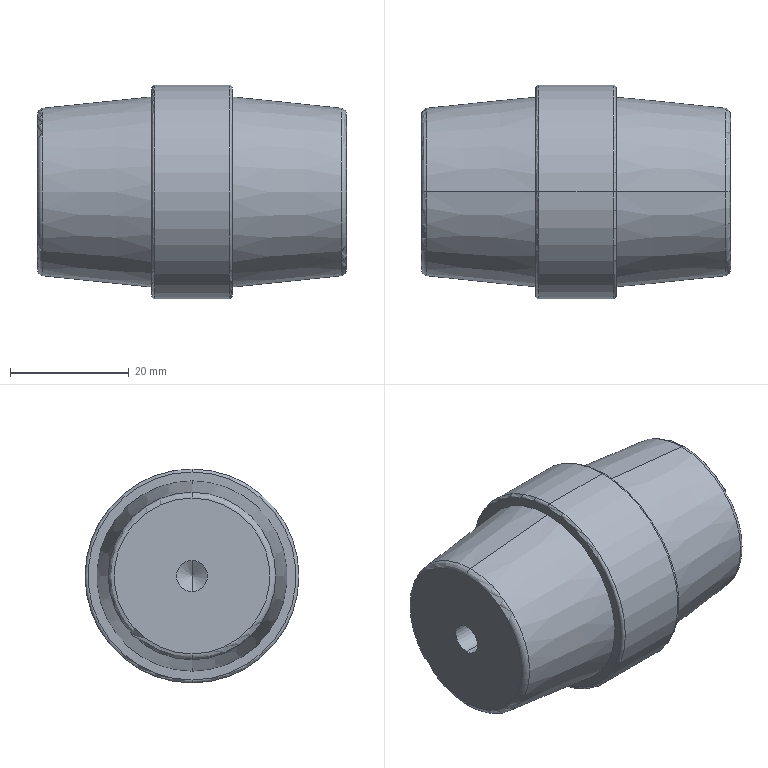Component | SolidWorks | InsulatorSYZ9-10Q100-1 | 1 solid | 26 faces | box 52 x 36 x 36 mm | volume 40423 mm3 | torus 8 | cone 8 | cylinder 6 | plane 4 | commonest cylinder face diameters 5.2 x4 36 x2
STEP:
#1=COLOUR_RGB('',0.7922,0.8196,0.9333);
#2=FILL_AREA_STYLE_COLOUR('',#1);
#3=FILL_AREA_STYLE('',(#2));
#4=SURFACE_STYLE_FILL_AREA(#3);
#5=SURFACE_SIDE_STYLE('',(#4));
#6=SURFACE_STYLE_USAGE(.BOTH.,#5);
#7=PRESENTATION_STYLE_ASSIGNMENT((#6));
#8=CARTESIAN_POINT('',(25.13,9.025,27.254));
#9=VERTEX_POINT('',#8);
#10=CARTESIAN_POINT('',(25.13,9.025,28.671));
#11=VERTEX_POINT('',#10);
#12=CARTESIAN_POINT('',(25.13,9.025,27.963));
#13=DIRECTION('',(1.,0.,0.));
#14=DIRECTION('',(0.,0.,1.));
#15=AXIS2_PLACEMENT_3D('',#12,#13,#14);
#16=CIRCLE('',#15,0.7087);
#17=EDGE_CURVE('',#9,#11,#16,.T.);
#18=ORIENTED_EDGE('',*,*,#17,.F.);
#19=CARTESIAN_POINT('',(25.11,9.025,27.274));
#20=VERTEX_POINT('',#19);
#21=CARTESIAN_POINT('',(25.13,9.025,27.274));
#22=DIRECTION('',(0.,1.,0.));
#23=DIRECTION('',(0.,0.,1.));
#24=AXIS2_PLACEMENT_3D('',#21,#22,#23);
#25=CIRCLE('',#24,0.01969);
#26=EDGE_CURVE('',#9,#20,#25,.T.);
#27=ORIENTED_EDGE('',*,*,#26,.T.);
#28=CARTESIAN_POINT('',(25.11,9.025,28.652));
#29=VERTEX_POINT('',#28);
#30=CARTESIAN_POINT('',(25.11,9.025,27.963));
#31=DIRECTION('',(-1.,0.,0.));
#32=DIRECTION('',(0.,0.,1.));
#33=AXIS2_PLACEMENT_3D('',#30,#31,#32);
#34=CIRCLE('',#33,0.689);
#35=EDGE_CURVE('',#29,#20,#34,.T.);
#36=ORIENTED_EDGE('',*,*,#35,.F.);
#37=CARTESIAN_POINT('',(25.13,9.025,28.652));
#38=DIRECTION('',(0.,-1.,0.));
#39=DIRECTION('',(0.,0.,-1.));
#40=AXIS2_PLACEMENT_3D('',#37,#38,#39);
#41=CIRCLE('',#40,0.01969);
#42=EDGE_CURVE('',#11,#29,#41,.T.);
#43=ORIENTED_EDGE('',*,*,#42,.F.);
#44=EDGE_LOOP('',(#18,#27,#36,#43));
#45=FACE_OUTER_BOUND('',#44,.T.);
#46=CARTESIAN_POINT('',(25.13,9.025,27.963));
#47=DIRECTION('',(-1.,0.,0.));
#48=DIRECTION('',(0.,0.,1.));
#49=AXIS2_PLACEMENT_3D('',#46,#47,#48);
#50=TOROIDAL_SURFACE('',#49,0.689,0.01969);
#51=ADVANCED_FACE('',(#45),#50,.T.);
#52=CARTESIAN_POINT('',(25.622,9.025,28.671));
#53=VERTEX_POINT('',#52);
#54=CARTESIAN_POINT('',(25.622,9.025,27.254));
#55=VERTEX_POINT('',#54);
#56=CARTESIAN_POINT('',(25.622,9.025,27.963));
#57=DIRECTION('',(-1.,0.,0.));
#58=DIRECTION('',(0.,0.,-1.));
#59=AXIS2_PLACEMENT_3D('',#56,#57,#58);
#60=CIRCLE('',#59,0.7087);
#61=EDGE_CURVE('',#53,#55,#60,.T.);
#62=ORIENTED_EDGE('',*,*,#61,.F.);
#63=CARTESIAN_POINT('',(25.642,9.025,28.652));
#64=VERTEX_POINT('',#63);
#65=CARTESIAN_POINT('',(25.622,9.025,28.652));
#66=DIRECTION('',(0.,1.,-0.));
#67=DIRECTION('',(0.,0.,1.));
#68=AXIS2_PLACEMENT_3D('',#65,#66,#67);
#69=CIRCLE('',#68,0.01969);
#70=EDGE_CURVE('',#53,#64,#69,.T.);
#71=ORIENTED_EDGE('',*,*,#70,.T.);
#72=CARTESIAN_POINT('',(25.642,9.025,27.274));
#73=VERTEX_POINT('',#72);
#74=CARTESIAN_POINT('',(25.642,9.025,27.963));
#75=DIRECTION('',(1.,0.,0.));
#76=DIRECTION('',(0.,0.,-1.));
#77=AXIS2_PLACEMENT_3D('',#74,#75,#76);
#78=CIRCLE('',#77,0.689);
#79=EDGE_CURVE('',#73,#64,#78,.T.);
#80=ORIENTED_EDGE('',*,*,#79,.F.);
#81=CARTESIAN_POINT('',(25.622,9.025,27.274));
#82=DIRECTION('',(0.,-1.,0.));
#83=DIRECTION('',(0.,0.,-1.));
#84=AXIS2_PLACEMENT_3D('',#81,#82,#83);
#85=CIRCLE('',#84,0.01969);
#86=EDGE_CURVE('',#55,#73,#85,.T.);
#87=ORIENTED_EDGE('',*,*,#86,.F.);
#88=EDGE_LOOP('',(#62,#71,#80,#87));
#89=FACE_OUTER_BOUND('',#88,.T.);
#90=CARTESIAN_POINT('',(25.622,9.025,27.963));
#91=DIRECTION('',(1.,0.,0.));
#92=DIRECTION('',(0.,0.,-1.));
#93=AXIS2_PLACEMENT_3D('',#90,#91,#92);
#94=TOROIDAL_SURFACE('',#93,0.689,0.01969);
#95=ADVANCED_FACE('',(#89),#94,.T.);
#96=CARTESIAN_POINT('',(24.388,9.025,27.408));
#97=VERTEX_POINT('',#96);
#98=CARTESIAN_POINT('',(24.388,9.025,28.517));
#99=VERTEX_POINT('',#98);
#100=CARTESIAN_POINT('',(24.388,9.025,27.963));
#101=DIRECTION('',(1.,0.,0.));
#102=DIRECTION('',(0.,0.,1.));
#103=AXIS2_PLACEMENT_3D('',#100,#101,#102);
#104=CIRCLE('',#103,0.5548);
#105=EDGE_CURVE('',#97,#99,#104,.T.);
#106=ORIENTED_EDGE('',*,*,#105,.F.);
#107=CARTESIAN_POINT('',(24.353,9.025,27.447));
#108=VERTEX_POINT('',#107);
#109=CARTESIAN_POINT('',(24.392,9.025,27.447));
#110=DIRECTION('',(0.,1.,0.));
#111=DIRECTION('',(0.,0.,1.));
#112=AXIS2_PLACEMENT_3D('',#109,#110,#111);
#113=CIRCLE('',#112,0.03937);
#114=EDGE_CURVE('',#97,#108,#113,.T.);
#115=ORIENTED_EDGE('',*,*,#114,.T.);
#116=CARTESIAN_POINT('',(24.353,9.025,28.478));
#117=VERTEX_POINT('',#116);
#118=CARTESIAN_POINT('',(24.353,9.025,27.963));
#119=DIRECTION('',(-1.,0.,0.));
#120=DIRECTION('',(0.,0.,1.));
#121=AXIS2_PLACEMENT_3D('',#118,#119,#120);
#122=CIRCLE('',#121,0.5157);
#123=EDGE_CURVE('',#117,#108,#122,.T.);
#124=ORIENTED_EDGE('',*,*,#123,.F.);
#125=CARTESIAN_POINT('',(24.392,9.025,28.478));
#126=DIRECTION('',(0.,-1.,0.));
#127=DIRECTION('',(0.,0.,-1.));
#128=AXIS2_PLACEMENT_3D('',#125,#126,#127);
#129=CIRCLE('',#128,0.03937);
#130=EDGE_CURVE('',#99,#117,#129,.T.);
#131=ORIENTED_EDGE('',*,*,#130,.F.);
#132=EDGE_LOOP('',(#106,#115,#124,#131));
#133=FACE_OUTER_BOUND('',#132,.T.);
#134=CARTESIAN_POINT('',(24.392,9.025,27.963));
#135=DIRECTION('',(-1.,0.,0.));
#136=DIRECTION('',(0.,0.,1.));
#137=AXIS2_PLACEMENT_3D('',#134,#135,#136);
#138=TOROIDAL_SURFACE('',#137,0.5157,0.03937);
#139=ADVANCED_FACE('',(#133),#138,.T.);
#140=CARTESIAN_POINT('',(26.364,9.025,28.517));
#141=VERTEX_POINT('',#140);
#142=CARTESIAN_POINT('',(26.364,9.025,27.408));
#143=VERTEX_POINT('',#142);
#144=CARTESIAN_POINT('',(26.364,9.025,27.963));
#145=DIRECTION('',(-1.,0.,0.));
#146=DIRECTION('',(0.,0.,-1.));
#147=AXIS2_PLACEMENT_3D('',#144,#145,#146);
#148=CIRCLE('',#147,0.5548);
#149=EDGE_CURVE('',#141,#143,#148,.T.);
#150=ORIENTED_EDGE('',*,*,#149,.F.);
#151=CARTESIAN_POINT('',(26.4,9.025,28.478));
#152=VERTEX_POINT('',#151);
#153=CARTESIAN_POINT('',(26.36,9.025,28.478));
#154=DIRECTION('',(0.,1.,-0.));
#155=DIRECTION('',(0.,0.,1.));
#156=AXIS2_PLACEMENT_3D('',#153,#154,#155);
#157=CIRCLE('',#156,0.03937);
#158=EDGE_CURVE('',#141,#152,#157,.T.);
#159=ORIENTED_EDGE('',*,*,#158,.T.);
#160=CARTESIAN_POINT('',(26.4,9.025,27.447));
#161=VERTEX_POINT('',#160);
#162=CARTESIAN_POINT('',(26.4,9.025,27.963));
#163=DIRECTION('',(1.,0.,0.));
#164=DIRECTION('',(0.,0.,-1.));
#165=AXIS2_PLACEMENT_3D('',#162,#163,#164);
#166=CIRCLE('',#165,0.5157);
#167=EDGE_CURVE('',#161,#152,#166,.T.);
#168=ORIENTED_EDGE('',*,*,#167,.F.);
#169=CARTESIAN_POINT('',(26.36,9.025,27.447));
#170=DIRECTION('',(0.,-1.,0.));
#171=DIRECTION('',(0.,0.,-1.));
#172=AXIS2_PLACEMENT_3D('',#169,#170,#171);
#173=CIRCLE('',#172,0.03937);
#174=EDGE_CURVE('',#143,#161,#173,.T.);
#175=ORIENTED_EDGE('',*,*,#174,.F.);
#176=EDGE_LOOP('',(#150,#159,#168,#175));
#177=FACE_OUTER_BOUND('',#176,.T.);
#178=CARTESIAN_POINT('',(26.36,9.025,27.963));
#179=DIRECTION('',(1.,0.,0.));
#180=DIRECTION('',(0.,0.,-1.));
#181=AXIS2_PLACEMENT_3D('',#178,#179,#180);
#182=TOROIDAL_SURFACE('',#181,0.5157,0.03937);
#183=ADVANCED_FACE('',(#177),#182,.T.);
#184=CARTESIAN_POINT('',(25.927,9.025,28.065));
#185=VERTEX_POINT('',#184);
#186=CARTESIAN_POINT('',(25.927,9.025,27.86));
#187=VERTEX_POINT('',#186);
#188=CARTESIAN_POINT('',(25.927,9.025,27.963));
#189=DIRECTION('',(1.,0.,0.));
#190=DIRECTION('',(0.,0.,-1.));
#191=AXIS2_PLACEMENT_3D('',#188,#189,#190);
#192=CIRCLE('',#191,0.1024);
#193=EDGE_CURVE('',#185,#187,#192,.T.);
#194=ORIENTED_EDGE('',*,*,#193,.F.);
#195=CARTESIAN_POINT('',(26.4,9.025,28.065));
#196=VERTEX_POINT('',#195);
#197=CARTESIAN_POINT('',(26.4,9.025,28.065));
#198=DIRECTION('',(1.,0.,0.));
#199=VECTOR('',#198,39.37);
#200=LINE('',#197,#199);
#201=EDGE_CURVE('',#185,#196,#200,.T.);
#202=ORIENTED_EDGE('',*,*,#201,.T.);
#203=CARTESIAN_POINT('',(26.4,9.025,27.86));
#204=VERTEX_POINT('',#203);
#205=CARTESIAN_POINT('',(26.4,9.025,27.963));
#206=DIRECTION('',(1.,0.,0.));
#207=DIRECTION('',(0.,0.,-1.));
#208=AXIS2_PLACEMENT_3D('',#205,#206,#207);
#209=CIRCLE('',#208,0.1024);
#210=EDGE_CURVE('',#196,#204,#209,.T.);
#211=ORIENTED_EDGE('',*,*,#210,.T.);
#212=CARTESIAN_POINT('',(26.4,9.025,27.86));
#213=DIRECTION('',(1.,0.,0.));
#214=VECTOR('',#213,39.37);
#215=LINE('',#212,#214);
#216=EDGE_CURVE('',#187,#204,#215,.T.);
#217=ORIENTED_EDGE('',*,*,#216,.F.);
#218=EDGE_LOOP('',(#194,#202,#211,#217));
#219=FACE_OUTER_BOUND('',#218,.T.);
#220=CARTESIAN_POINT('',(26.4,9.025,27.963));
#221=DIRECTION('',(1.,0.,0.));
#222=DIRECTION('',(0.,0.,-1.));
#223=AXIS2_PLACEMENT_3D('',#220,#221,#222);
#224=CYLINDRICAL_SURFACE('',#223,0.1024);
#225=ADVANCED_FACE('',(#219),#224,.F.);
#226=CARTESIAN_POINT('',(25.866,9.025,27.963));
#227=VERTEX_POINT('',#226);
#228=CARTESIAN_POINT('',(25.927,9.025,27.86));
#229=DIRECTION('',(0.515,0.,-0.8572));
#230=VECTOR('',#229,39.37);
#231=LINE('',#228,#230);
#232=EDGE_CURVE('',#227,#187,#231,.T.);
#233=ORIENTED_EDGE('',*,*,#232,.F.);
#234=CARTESIAN_POINT('',(25.927,9.025,28.065));
#235=DIRECTION('',(0.515,0.,0.8572));
#236=VECTOR('',#235,39.37);
#237=LINE('',#234,#236);
#238=EDGE_CURVE('',#227,#185,#237,.T.);
#239=ORIENTED_EDGE('',*,*,#238,.T.);
#240=ORIENTED_EDGE('',*,*,#193,.T.);
#241=EDGE_LOOP('',(#233,#239,#240));
#242=FACE_OUTER_BOUND('',#241,.T.);
#243=CARTESIAN_POINT('',(25.927,9.025,27.963));
#244=DIRECTION('',(1.,0.,0.));
#245=DIRECTION('',(0.,0.,-1.));
#246=AXIS2_PLACEMENT_3D('',#243,#244,#245);
#247=CONICAL_SURFACE('',#246,0.1024,1.03);
#248=ADVANCED_FACE('',(#242),#247,.F.);
#249=CARTESIAN_POINT('',(26.364,9.025,27.963));
#250=DIRECTION('',(-1.,0.,0.));
#251=DIRECTION('',(0.,0.,-1.));
#252=AXIS2_PLACEMENT_3D('',#249,#250,#251);
#253=CIRCLE('',#252,0.5548);
#254=EDGE_CURVE('',#143,#141,#253,.T.);
#255=ORIENTED_EDGE('',*,*,#254,.T.);
#256=CARTESIAN_POINT('',(25.642,9.025,28.593));
#257=VERTEX_POINT('',#256);
#258=CARTESIAN_POINT('',(26.4,9.025,28.514));
#259=DIRECTION('',(-0.9946,-0.,0.1033));
#260=VECTOR('',#259,39.37);
#261=LINE('',#258,#260);
#262=EDGE_CURVE('',#141,#257,#261,.T.);
#263=ORIENTED_EDGE('',*,*,#262,.T.);
#264=CARTESIAN_POINT('',(25.642,9.025,27.333));
#265=VERTEX_POINT('',#264);
#266=CARTESIAN_POINT('',(25.642,9.025,27.963));
#267=DIRECTION('',(-1.,0.,0.));
#268=DIRECTION('',(0.,0.,1.));
#269=AXIS2_PLACEMENT_3D('',#266,#267,#268);
#270=CIRCLE('',#269,0.6299);
#271=EDGE_CURVE('',#265,#257,#270,.T.);
#272=ORIENTED_EDGE('',*,*,#271,.F.);
#273=CARTESIAN_POINT('',(26.4,9.025,27.411));
#274=DIRECTION('',(-0.9946,0.,-0.1033));
#275=VECTOR('',#274,39.37);
#276=LINE('',#273,#275);
#277=EDGE_CURVE('',#143,#265,#276,.T.);
#278=ORIENTED_EDGE('',*,*,#277,.F.);
#279=EDGE_LOOP('',(#255,#263,#272,#278));
#280=FACE_OUTER_BOUND('',#279,.T.);
#281=CARTESIAN_POINT('',(26.4,9.025,27.963));
#282=DIRECTION('',(-1.,0.,0.));
#283=DIRECTION('',(0.,0.,-1.));
#284=AXIS2_PLACEMENT_3D('',#281,#282,#283);
#285=CONICAL_SURFACE('',#284,0.5512,0.1035);
#286=ADVANCED_FACE('',(#280),#285,.T.);
#287=CARTESIAN_POINT('',(24.825,9.025,27.86));
#288=VERTEX_POINT('',#287);
#289=CARTESIAN_POINT('',(24.825,9.025,28.065));
#290=VERTEX_POINT('',#289);
#291=CARTESIAN_POINT('',(24.825,9.025,27.963));
#292=DIRECTION('',(-1.,0.,0.));
#293=DIRECTION('',(0.,0.,1.));
#294=AXIS2_PLACEMENT_3D('',#291,#292,#293);
#295=CIRCLE('',#294,0.1024);
#296=EDGE_CURVE('',#288,#290,#295,.T.);
#297=ORIENTED_EDGE('',*,*,#296,.F.);
#298=CARTESIAN_POINT('',(24.353,9.025,27.86));
#299=VERTEX_POINT('',#298);
#300=CARTESIAN_POINT('',(24.353,9.025,27.86));
#301=DIRECTION('',(-1.,0.,0.));
#302=VECTOR('',#301,39.37);
#303=LINE('',#300,#302);
#304=EDGE_CURVE('',#288,#299,#303,.T.);
#305=ORIENTED_EDGE('',*,*,#304,.T.);
#306=CARTESIAN_POINT('',(24.353,9.025,28.065));
#307=VERTEX_POINT('',#306);
#308=CARTESIAN_POINT('',(24.353,9.025,27.963));
#309=DIRECTION('',(-1.,0.,0.));
#310=DIRECTION('',(0.,0.,1.));
#311=AXIS2_PLACEMENT_3D('',#308,#309,#310);
#312=CIRCLE('',#311,0.1024);
#313=EDGE_CURVE('',#299,#307,#312,.T.);
#314=ORIENTED_EDGE('',*,*,#313,.T.);
#315=CARTESIAN_POINT('',(24.353,9.025,28.065));
#316=DIRECTION('',(-1.,0.,0.));
#317=VECTOR('',#316,39.37);
#318=LINE('',#315,#317);
#319=EDGE_CURVE('',#290,#307,#318,.T.);
#320=ORIENTED_EDGE('',*,*,#319,.F.);
#321=EDGE_LOOP('',(#297,#305,#314,#320));
#322=FACE_OUTER_BOUND('',#321,.T.);
#323=CARTESIAN_POINT('',(24.353,9.025,27.963));
#324=DIRECTION('',(-1.,0.,0.));
#325=DIRECTION('',(0.,0.,1.));
#326=AXIS2_PLACEMENT_3D('',#323,#324,#325);
#327=CYLINDRICAL_SURFACE('',#326,0.1024);
#328=ADVANCED_FACE('',(#322),#327,.F.);
#329=CARTESIAN_POINT('',(24.886,9.025,27.963));
#330=VERTEX_POINT('',#329);
#331=CARTESIAN_POINT('',(24.825,9.025,28.065));
#332=DIRECTION('',(-0.515,0.,0.8572));
#333=VECTOR('',#332,39.37);
#334=LINE('',#331,#333);
#335=EDGE_CURVE('',#330,#290,#334,.T.);
#336=ORIENTED_EDGE('',*,*,#335,.F.);
#337=CARTESIAN_POINT('',(24.825,9.025,27.86));
#338=DIRECTION('',(-0.515,0.,-0.8572));
#339=VECTOR('',#338,39.37);
#340=LINE('',#337,#339);
#341=EDGE_CURVE('',#330,#288,#340,.T.);
#342=ORIENTED_EDGE('',*,*,#341,.T.);
#343=ORIENTED_EDGE('',*,*,#296,.T.);
#344=EDGE_LOOP('',(#336,#342,#343));
#345=FACE_OUTER_BOUND('',#344,.T.);
#346=CARTESIAN_POINT('',(24.825,9.025,27.963));
#347=DIRECTION('',(-1.,0.,0.));
#348=DIRECTION('',(0.,0.,1.));
#349=AXIS2_PLACEMENT_3D('',#346,#347,#348);
#350=CONICAL_SURFACE('',#349,0.1024,1.03);
#351=ADVANCED_FACE('',(#345),#350,.F.);
#352=ORIENTED_EDGE('',*,*,#61,.T.);
#353=CARTESIAN_POINT('',(24.353,9.025,27.254));
#354=DIRECTION('',(-1.,0.,0.));
#355=VECTOR('',#354,39.37);
#356=LINE('',#353,#355);
#357=EDGE_CURVE('',#55,#9,#356,.T.);
#358=ORIENTED_EDGE('',*,*,#357,.T.);
#359=ORIENTED_EDGE('',*,*,#17,.T.);
#360=CARTESIAN_POINT('',(24.353,9.025,28.671));
#361=DIRECTION('',(-1.,0.,0.));
#362=VECTOR('',#361,39.37);
#363=LINE('',#360,#362);
#364=EDGE_CURVE('',#53,#11,#363,.T.);
#365=ORIENTED_EDGE('',*,*,#364,.F.);
#366=EDGE_LOOP('',(#352,#358,#359,#365));
#367=FACE_OUTER_BOUND('',#366,.T.);
#368=CARTESIAN_POINT('',(24.353,9.025,27.963));
#369=DIRECTION('',(-1.,0.,0.));
#370=DIRECTION('',(0.,0.,1.));
#371=AXIS2_PLACEMENT_3D('',#368,#369,#370);
#372=CYLINDRICAL_SURFACE('',#371,0.7087);
#373=ADVANCED_FACE('',(#367),#372,.T.);
#374=ORIENTED_EDGE('',*,*,#105,.T.);
#375=CARTESIAN_POINT('',(25.11,9.025,28.593));
#376=VERTEX_POINT('',#375);
#377=CARTESIAN_POINT('',(24.353,9.025,28.514));
#378=DIRECTION('',(0.9946,0.,0.1033));
#379=VECTOR('',#378,39.37);
#380=LINE('',#377,#379);
#381=EDGE_CURVE('',#99,#376,#380,.T.);
#382=ORIENTED_EDGE('',*,*,#381,.T.);
#383=CARTESIAN_POINT('',(25.11,9.025,27.333));
#384=VERTEX_POINT('',#383);
#385=CARTESIAN_POINT('',(25.11,9.025,27.963));
#386=DIRECTION('',(-1.,0.,0.));
#387=DIRECTION('',(0.,0.,1.));
#388=AXIS2_PLACEMENT_3D('',#385,#386,#387);
#389=CIRCLE('',#388,0.6299);
#390=EDGE_CURVE('',#376,#384,#389,.T.);
#391=ORIENTED_EDGE('',*,*,#390,.T.);
#392=CARTESIAN_POINT('',(24.353,9.025,27.411));
#393=DIRECTION('',(0.9946,0.,-0.1033));
#394=VECTOR('',#393,39.37);
#395=LINE('',#392,#394);
#396=EDGE_CURVE('',#97,#384,#395,.T.);
#397=ORIENTED_EDGE('',*,*,#396,.F.);
#398=EDGE_LOOP('',(#374,#382,#391,#397));
#399=FACE_OUTER_BOUND('',#398,.T.);
#400=CARTESIAN_POINT('',(24.353,9.025,27.963));
#401=DIRECTION('',(1.,0.,0.));
#402=DIRECTION('',(0.,0.,-1.));
#403=AXIS2_PLACEMENT_3D('',#400,#401,#402);
#404=CONICAL_SURFACE('',#403,0.5512,0.1035);
#405=ADVANCED_FACE('',(#399),#404,.T.);
#406=ORIENTED_EDGE('',*,*,#123,.T.);
#407=CARTESIAN_POINT('',(24.353,9.025,27.963));
#408=DIRECTION('',(-1.,0.,0.));
#409=DIRECTION('',(0.,0.,1.));
#410=AXIS2_PLACEMENT_3D('',#407,#408,#409);
#411=CIRCLE('',#410,0.5157);
#412=EDGE_CURVE('',#108,#117,#411,.T.);
#413=ORIENTED_EDGE('',*,*,#412,.T.);
#414=EDGE_LOOP('',(#406,#413));
#415=FACE_OUTER_BOUND('',#414,.T.);
#416=CARTESIAN_POINT('',(24.353,9.025,27.963));
#417=DIRECTION('',(-1.,0.,0.));
#418=DIRECTION('',(0.,0.,1.));
#419=AXIS2_PLACEMENT_3D('',#416,#417,#418);
#420=CIRCLE('',#419,0.1024);
#421=EDGE_CURVE('',#307,#299,#420,.T.);
#422=ORIENTED_EDGE('',*,*,#421,.F.);
#423=ORIENTED_EDGE('',*,*,#313,.F.);
#424=EDGE_LOOP('',(#422,#423));
#425=FACE_BOUND('',#424,.T.);
#426=CARTESIAN_POINT('',(24.353,9.025,27.963));
#427=DIRECTION('',(-1.,0.,0.));
#428=DIRECTION('',(0.,0.,1.));
#429=AXIS2_PLACEMENT_3D('',#426,#427,#428);
#430=PLANE('',#429);
#431=ADVANCED_FACE('',(#415,#425),#430,.T.);
#432=ORIENTED_EDGE('',*,*,#381,.F.);
#433=CARTESIAN_POINT('',(24.388,9.025,27.963));
#434=DIRECTION('',(1.,0.,0.));
#435=DIRECTION('',(0.,0.,1.));
#436=AXIS2_PLACEMENT_3D('',#433,#434,#435);
#437=CIRCLE('',#436,0.5548);
#438=EDGE_CURVE('',#99,#97,#437,.T.);
#439=ORIENTED_EDGE('',*,*,#438,.T.);
#440=ORIENTED_EDGE('',*,*,#396,.T.);
#441=CARTESIAN_POINT('',(25.11,9.025,27.963));
#442=DIRECTION('',(-1.,0.,0.));
#443=DIRECTION('',(0.,0.,1.));
#444=AXIS2_PLACEMENT_3D('',#441,#442,#443);
#445=CIRCLE('',#444,0.6299);
#446=EDGE_CURVE('',#384,#376,#445,.T.);
#447=ORIENTED_EDGE('',*,*,#446,.T.);
#448=EDGE_LOOP('',(#432,#439,#440,#447));
#449=FACE_OUTER_BOUND('',#448,.T.);
#450=CARTESIAN_POINT('',(24.353,9.025,27.963));
#451=DIRECTION('',(1.,0.,0.));
#452=DIRECTION('',(0.,0.,-1.));
#453=AXIS2_PLACEMENT_3D('',#450,#451,#452);
#454=CONICAL_SURFACE('',#453,0.5512,0.1035);
#455=ADVANCED_FACE('',(#449),#454,.T.);
#456=ORIENTED_EDGE('',*,*,#35,.T.);
#457=CARTESIAN_POINT('',(25.11,9.025,27.963));
#458=DIRECTION('',(-1.,0.,0.));
#459=DIRECTION('',(0.,0.,1.));
#460=AXIS2_PLACEMENT_3D('',#457,#458,#459);
#461=CIRCLE('',#460,0.689);
#462=EDGE_CURVE('',#20,#29,#461,.T.);
#463=ORIENTED_EDGE('',*,*,#462,.T.);
#464=EDGE_LOOP('',(#456,#463));
#465=FACE_OUTER_BOUND('',#464,.T.);
#466=ORIENTED_EDGE('',*,*,#446,.F.);
#467=ORIENTED_EDGE('',*,*,#390,.F.);
#468=EDGE_LOOP('',(#466,#467));
#469=FACE_BOUND('',#468,.T.);
#470=CARTESIAN_POINT('',(25.11,8.395,27.963));
#471=DIRECTION('',(-1.,0.,0.));
#472=DIRECTION('',(0.,0.,1.));
#473=AXIS2_PLACEMENT_3D('',#470,#471,#472);
#474=PLANE('',#473);
#475=ADVANCED_FACE('',(#465,#469),#474,.T.);
#476=ORIENTED_EDGE('',*,*,#357,.F.);
#477=CARTESIAN_POINT('',(25.622,9.025,27.963));
#478=DIRECTION('',(-1.,0.,0.));
#479=DIRECTION('',(0.,0.,-1.));
#480=AXIS2_PLACEMENT_3D('',#477,#478,#479);
#481=CIRCLE('',#480,0.7087);
#482=EDGE_CURVE('',#55,#53,#481,.T.);
#483=ORIENTED_EDGE('',*,*,#482,.T.);
#484=ORIENTED_EDGE('',*,*,#364,.T.);
#485=CARTESIAN_POINT('',(25.13,9.025,27.963));
#486=DIRECTION('',(1.,0.,0.));
#487=DIRECTION('',(0.,0.,1.));
#488=AXIS2_PLACEMENT_3D('',#485,#486,#487);
#489=CIRCLE('',#488,0.7087);
#490=EDGE_CURVE('',#11,#9,#489,.T.);
#491=ORIENTED_EDGE('',*,*,#490,.T.);
#492=EDGE_LOOP('',(#476,#483,#484,#491));
#493=FACE_OUTER_BOUND('',#492,.T.);
#494=CARTESIAN_POINT('',(24.353,9.025,27.963));
#495=DIRECTION('',(-1.,0.,0.));
#496=DIRECTION('',(0.,0.,1.));
#497=AXIS2_PLACEMENT_3D('',#494,#495,#496);
#498=CYLINDRICAL_SURFACE('',#497,0.7087);
#499=ADVANCED_FACE('',(#493),#498,.T.);
#500=ORIENTED_EDGE('',*,*,#341,.F.);
#501=ORIENTED_EDGE('',*,*,#335,.T.);
#502=CARTESIAN_POINT('',(24.825,9.025,27.963));
#503=DIRECTION('',(-1.,0.,0.));
#504=DIRECTION('',(0.,0.,1.));
#505=AXIS2_PLACEMENT_3D('',#502,#503,#504);
#506=CIRCLE('',#505,0.1024);
#507=EDGE_CURVE('',#290,#288,#506,.T.);
#508=ORIENTED_EDGE('',*,*,#507,.T.);
#509=EDGE_LOOP('',(#500,#501,#508));
#510=FACE_OUTER_BOUND('',#509,.T.);
#511=CARTESIAN_POINT('',(24.825,9.025,27.963));
#512=DIRECTION('',(-1.,0.,0.));
#513=DIRECTION('',(0.,0.,1.));
#514=AXIS2_PLACEMENT_3D('',#511,#512,#513);
#515=CONICAL_SURFACE('',#514,0.1024,1.03);
#516=ADVANCED_FACE('',(#510),#515,.F.);
#517=ORIENTED_EDGE('',*,*,#304,.F.);
#518=ORIENTED_EDGE('',*,*,#507,.F.);
#519=ORIENTED_EDGE('',*,*,#319,.T.);
#520=ORIENTED_EDGE('',*,*,#421,.T.);
#521=EDGE_LOOP('',(#517,#518,#519,#520));
#522=FACE_OUTER_BOUND('',#521,.T.);
#523=CARTESIAN_POINT('',(24.353,9.025,27.963));
#524=DIRECTION('',(-1.,0.,0.));
#525=DIRECTION('',(0.,0.,1.));
#526=AXIS2_PLACEMENT_3D('',#523,#524,#525);
#527=CYLINDRICAL_SURFACE('',#526,0.1024);
#528=ADVANCED_FACE('',(#522),#527,.F.);
#529=ORIENTED_EDGE('',*,*,#167,.T.);
#530=CARTESIAN_POINT('',(26.4,9.025,27.963));
#531=DIRECTION('',(1.,0.,0.));
#532=DIRECTION('',(0.,0.,-1.));
#533=AXIS2_PLACEMENT_3D('',#530,#531,#532);
#534=CIRCLE('',#533,0.5157);
#535=EDGE_CURVE('',#152,#161,#534,.T.);
#536=ORIENTED_EDGE('',*,*,#535,.T.);
#537=EDGE_LOOP('',(#529,#536));
#538=FACE_OUTER_BOUND('',#537,.T.);
#539=CARTESIAN_POINT('',(26.4,9.025,27.963));
#540=DIRECTION('',(1.,0.,0.));
#541=DIRECTION('',(0.,0.,-1.));
#542=AXIS2_PLACEMENT_3D('',#539,#540,#541);
#543=CIRCLE('',#542,0.1024);
#544=EDGE_CURVE('',#204,#196,#543,.T.);
#545=ORIENTED_EDGE('',*,*,#544,.F.);
#546=ORIENTED_EDGE('',*,*,#210,.F.);
#547=EDGE_LOOP('',(#545,#546));
#548=FACE_BOUND('',#547,.T.);
#549=CARTESIAN_POINT('',(26.4,9.025,27.963));
#550=DIRECTION('',(1.,0.,0.));
#551=DIRECTION('',(0.,0.,1.));
#552=AXIS2_PLACEMENT_3D('',#549,#550,#551);
#553=PLANE('',#552);
#554=ADVANCED_FACE('',(#538,#548),#553,.T.);
#555=ORIENTED_EDGE('',*,*,#262,.F.);
#556=ORIENTED_EDGE('',*,*,#149,.T.);
#557=ORIENTED_EDGE('',*,*,#277,.T.);
#558=CARTESIAN_POINT('',(25.642,9.025,27.963));
#559=DIRECTION('',(-1.,0.,0.));
#560=DIRECTION('',(0.,0.,1.));
#561=AXIS2_PLACEMENT_3D('',#558,#559,#560);
#562=CIRCLE('',#561,0.6299);
#563=EDGE_CURVE('',#257,#265,#562,.T.);
#564=ORIENTED_EDGE('',*,*,#563,.F.);
#565=EDGE_LOOP('',(#555,#556,#557,#564));
#566=FACE_OUTER_BOUND('',#565,.T.);
#567=CARTESIAN_POINT('',(26.4,9.025,27.963));
#568=DIRECTION('',(-1.,0.,0.));
#569=DIRECTION('',(0.,0.,-1.));
#570=AXIS2_PLACEMENT_3D('',#567,#568,#569);
#571=CONICAL_SURFACE('',#570,0.5512,0.1035);
#572=ADVANCED_FACE('',(#566),#571,.T.);
#573=ORIENTED_EDGE('',*,*,#79,.T.);
#574=CARTESIAN_POINT('',(25.642,9.025,27.963));
#575=DIRECTION('',(1.,0.,0.));
#576=DIRECTION('',(0.,0.,-1.));
#577=AXIS2_PLACEMENT_3D('',#574,#575,#576);
#578=CIRCLE('',#577,0.689);
#579=EDGE_CURVE('',#64,#73,#578,.T.);
#580=ORIENTED_EDGE('',*,*,#579,.T.);
#581=EDGE_LOOP('',(#573,#580));
#582=FACE_OUTER_BOUND('',#581,.T.);
#583=ORIENTED_EDGE('',*,*,#271,.T.);
#584=ORIENTED_EDGE('',*,*,#563,.T.);
#585=EDGE_LOOP('',(#583,#584));
#586=FACE_BOUND('',#585,.T.);
#587=CARTESIAN_POINT('',(25.642,8.395,27.963));
#588=DIRECTION('',(1.,0.,0.));
#589=DIRECTION('',(0.,0.,1.));
#590=AXIS2_PLACEMENT_3D('',#587,#588,#589);
#591=PLANE('',#590);
#592=ADVANCED_FACE('',(#582,#586),#591,.T.);
#593=ORIENTED_EDGE('',*,*,#238,.F.);
#594=ORIENTED_EDGE('',*,*,#232,.T.);
#595=CARTESIAN_POINT('',(25.927,9.025,27.963));
#596=DIRECTION('',(1.,0.,0.));
#597=DIRECTION('',(0.,0.,-1.));
#598=AXIS2_PLACEMENT_3D('',#595,#596,#597);
#599=CIRCLE('',#598,0.1024);
#600=EDGE_CURVE('',#187,#185,#599,.T.);
#601=ORIENTED_EDGE('',*,*,#600,.T.);
#602=EDGE_LOOP('',(#593,#594,#601));
#603=FACE_OUTER_BOUND('',#602,.T.);
#604=CARTESIAN_POINT('',(25.927,9.025,27.963));
#605=DIRECTION('',(1.,0.,0.));
#606=DIRECTION('',(0.,0.,-1.));
#607=AXIS2_PLACEMENT_3D('',#604,#605,#606);
#608=CONICAL_SURFACE('',#607,0.1024,1.03);
#609=ADVANCED_FACE('',(#603),#608,.F.);
#610=ORIENTED_EDGE('',*,*,#201,.F.);
#611=ORIENTED_EDGE('',*,*,#600,.F.);
#612=ORIENTED_EDGE('',*,*,#216,.T.);
#613=ORIENTED_EDGE('',*,*,#544,.T.);
#614=EDGE_LOOP('',(#610,#611,#612,#613));
#615=FACE_OUTER_BOUND('',#614,.T.);
#616=CARTESIAN_POINT('',(26.4,9.025,27.963));
#617=DIRECTION('',(1.,0.,0.));
#618=DIRECTION('',(0.,0.,-1.));
#619=AXIS2_PLACEMENT_3D('',#616,#617,#618);
#620=CYLINDRICAL_SURFACE('',#619,0.1024);
#621=ADVANCED_FACE('',(#615),#620,.F.);
#622=ORIENTED_EDGE('',*,*,#158,.F.);
#623=ORIENTED_EDGE('',*,*,#254,.F.);
#624=ORIENTED_EDGE('',*,*,#174,.T.);
#625=ORIENTED_EDGE('',*,*,#535,.F.);
#626=EDGE_LOOP('',(#622,#623,#624,#625));
#627=FACE_OUTER_BOUND('',#626,.T.);
#628=CARTESIAN_POINT('',(26.36,9.025,27.963));
#629=DIRECTION('',(1.,0.,0.));
#630=DIRECTION('',(0.,0.,-1.));
#631=AXIS2_PLACEMENT_3D('',#628,#629,#630);
#632=TOROIDAL_SURFACE('',#631,0.5157,0.03937);
#633=ADVANCED_FACE('',(#627),#632,.T.);
#634=ORIENTED_EDGE('',*,*,#114,.F.);
#635=ORIENTED_EDGE('',*,*,#438,.F.);
#636=ORIENTED_EDGE('',*,*,#130,.T.);
#637=ORIENTED_EDGE('',*,*,#412,.F.);
#638=EDGE_LOOP('',(#634,#635,#636,#637));
#639=FACE_OUTER_BOUND('',#638,.T.);
#640=CARTESIAN_POINT('',(24.392,9.025,27.963));
#641=DIRECTION('',(-1.,0.,0.));
#642=DIRECTION('',(0.,0.,1.));
#643=AXIS2_PLACEMENT_3D('',#640,#641,#642);
#644=TOROIDAL_SURFACE('',#643,0.5157,0.03937);
#645=ADVANCED_FACE('',(#639),#644,.T.);
#646=ORIENTED_EDGE('',*,*,#70,.F.);
#647=ORIENTED_EDGE('',*,*,#482,.F.);
#648=ORIENTED_EDGE('',*,*,#86,.T.);
#649=ORIENTED_EDGE('',*,*,#579,.F.);
#650=EDGE_LOOP('',(#646,#647,#648,#649));
#651=FACE_OUTER_BOUND('',#650,.T.);
#652=CARTESIAN_POINT('',(25.622,9.025,27.963));
#653=DIRECTION('',(1.,0.,0.));
#654=DIRECTION('',(0.,0.,-1.));
#655=AXIS2_PLACEMENT_3D('',#652,#653,#654);
#656=TOROIDAL_SURFACE('',#655,0.689,0.01969);
#657=ADVANCED_FACE('',(#651),#656,.T.);
#658=ORIENTED_EDGE('',*,*,#26,.F.);
#659=ORIENTED_EDGE('',*,*,#490,.F.);
#660=ORIENTED_EDGE('',*,*,#42,.T.);
#661=ORIENTED_EDGE('',*,*,#462,.F.);
#662=EDGE_LOOP('',(#658,#659,#660,#661));
#663=FACE_OUTER_BOUND('',#662,.T.);
#664=CARTESIAN_POINT('',(25.13,9.025,27.963));
#665=DIRECTION('',(-1.,0.,0.));
#666=DIRECTION('',(0.,0.,1.));
#667=AXIS2_PLACEMENT_3D('',#664,#665,#666);
#668=TOROIDAL_SURFACE('',#667,0.689,0.01969);
#669=ADVANCED_FACE('',(#663),#668,.T.);
#670=CLOSED_SHELL('',(#51,#95,#139,#183,#225,#248,#286,#328,#351,#373,#405,#431,#455,#475,#499,#516,#528,#554,#572,#592,#609,#621,#633,#645,#657,#669));
#671=MANIFOLD_SOLID_BREP('',#670);
#672=STYLED_ITEM('',(#7),#671);
#673=PRESENTATION_LAYER_ASSIGNMENT('','',(#672));
#674=(LENGTH_UNIT()NAMED_UNIT(*)SI_UNIT($,.METRE.));
#675=LENGTH_MEASURE_WITH_UNIT(LENGTH_MEASURE(0.0254),#674);
#676=DIMENSIONAL_EXPONENTS(1.,0.,0.,0.,0.,0.,0.);
#677=(CONVERSION_BASED_UNIT('',#675)LENGTH_UNIT()NAMED_UNIT(#676));
#678=UNCERTAINTY_MEASURE_WITH_UNIT(LENGTH_MEASURE(0.00001),#677,'','');
#679=(NAMED_UNIT(*)PLANE_ANGLE_UNIT()SI_UNIT($,.RADIAN.));
#680=(NAMED_UNIT(*)SI_UNIT($,.STERADIAN.)SOLID_ANGLE_UNIT());
#681=(GEOMETRIC_REPRESENTATION_CONTEXT(3)GLOBAL_UNCERTAINTY_ASSIGNED_CONTEXT((#678))GLOBAL_UNIT_ASSIGNED_CONTEXT((#677,#679,#680))REPRESENTATION_CONTEXT('',''));
#682=MECHANICAL_DESIGN_GEOMETRIC_PRESENTATION_REPRESENTATION('',(#672),#681);
#683=CARTESIAN_POINT('',(0.,0.,0.));
#684=DIRECTION('',(0.,0.,1.));
#685=DIRECTION('',(1.,0.,0.));
#686=AXIS2_PLACEMENT_3D('',#683,#684,#685);
#687=(LENGTH_UNIT()NAMED_UNIT(*)SI_UNIT($,.METRE.));
#688=LENGTH_MEASURE_WITH_UNIT(LENGTH_MEASURE(0.0254),#687);
#689=DIMENSIONAL_EXPONENTS(1.,0.,0.,0.,0.,0.,0.);
#690=(CONVERSION_BASED_UNIT('',#688)LENGTH_UNIT()NAMED_UNIT(#689));
#691=UNCERTAINTY_MEASURE_WITH_UNIT(LENGTH_MEASURE(0.00001),#690,'','');
#692=(NAMED_UNIT(*)PLANE_ANGLE_UNIT()SI_UNIT($,.RADIAN.));
#693=(NAMED_UNIT(*)SI_UNIT($,.STERADIAN.)SOLID_ANGLE_UNIT());
#694=(GEOMETRIC_REPRESENTATION_CONTEXT(3)GLOBAL_UNCERTAINTY_ASSIGNED_CONTEXT((#691))GLOBAL_UNIT_ASSIGNED_CONTEXT((#690,#692,#693))REPRESENTATION_CONTEXT('',''));
#695=ADVANCED_BREP_SHAPE_REPRESENTATION('',(#671,#686),#694);